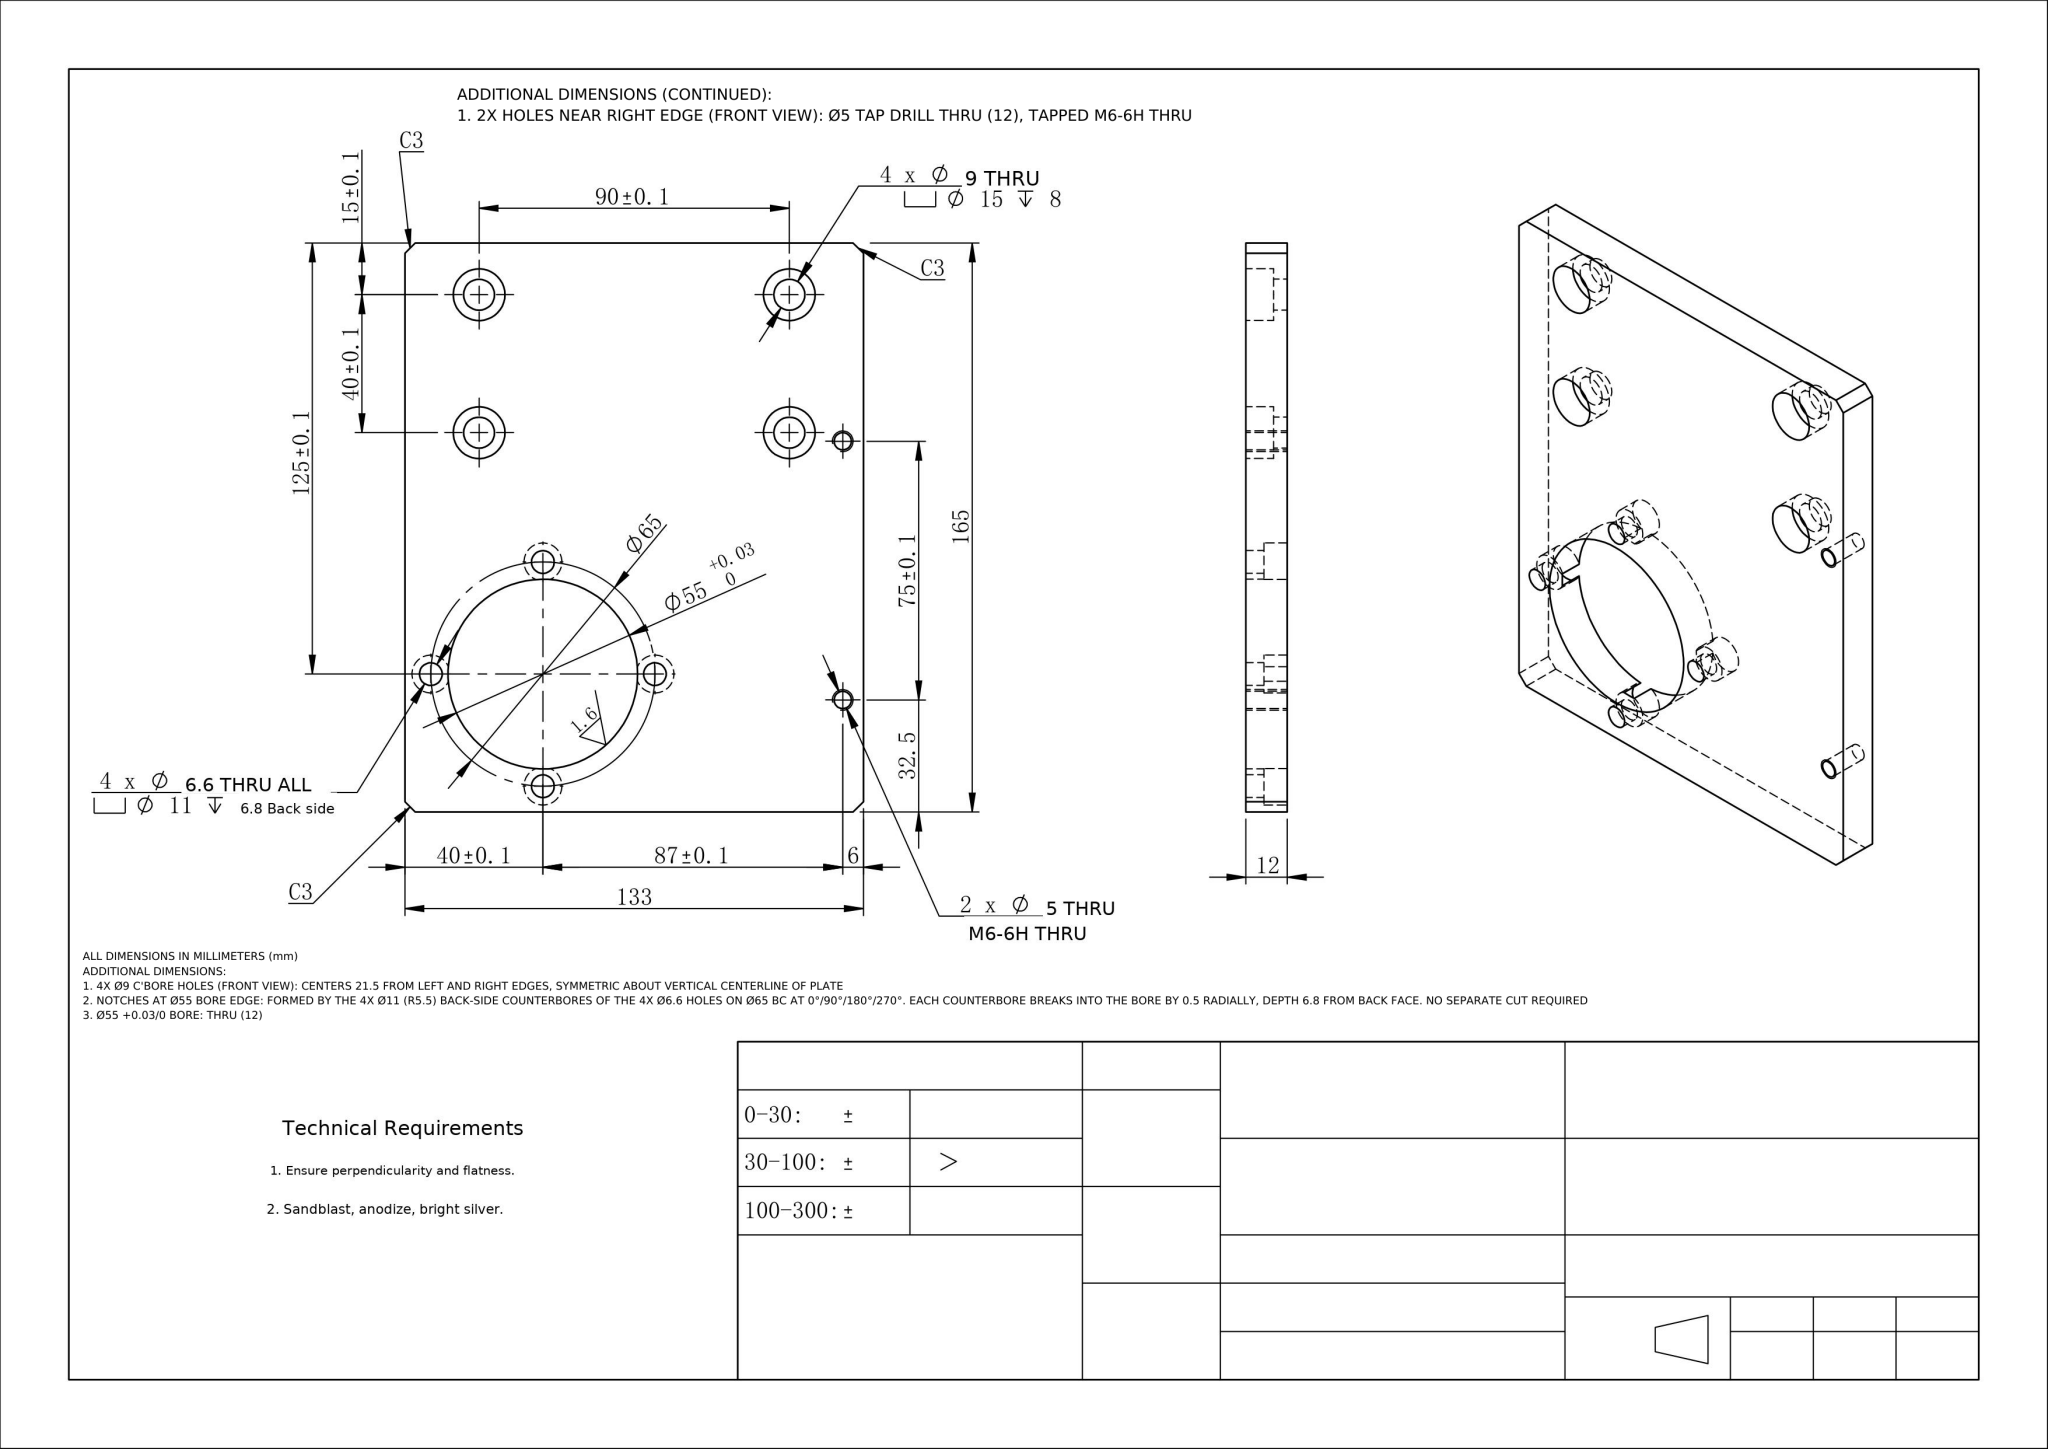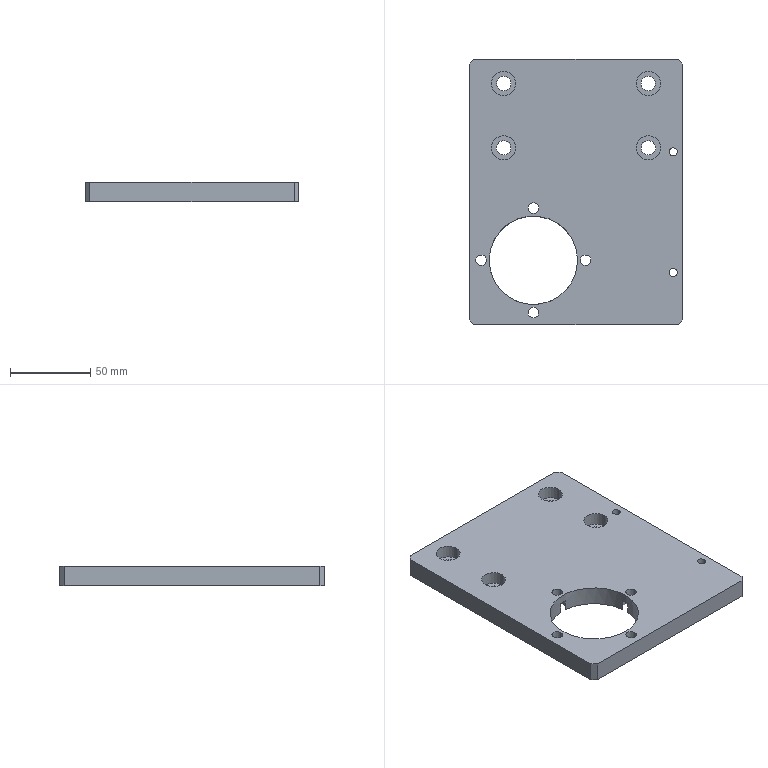Part | NX | mm | 1 solid | 57 faces | box 133 x 165 x 12 mm | volume 224212 mm3 | cylinder 39 | plane 18 | commonest cylinder face diameters 11 x9 6.6 x8 15 x8 9 x8 5 x4 55 x2